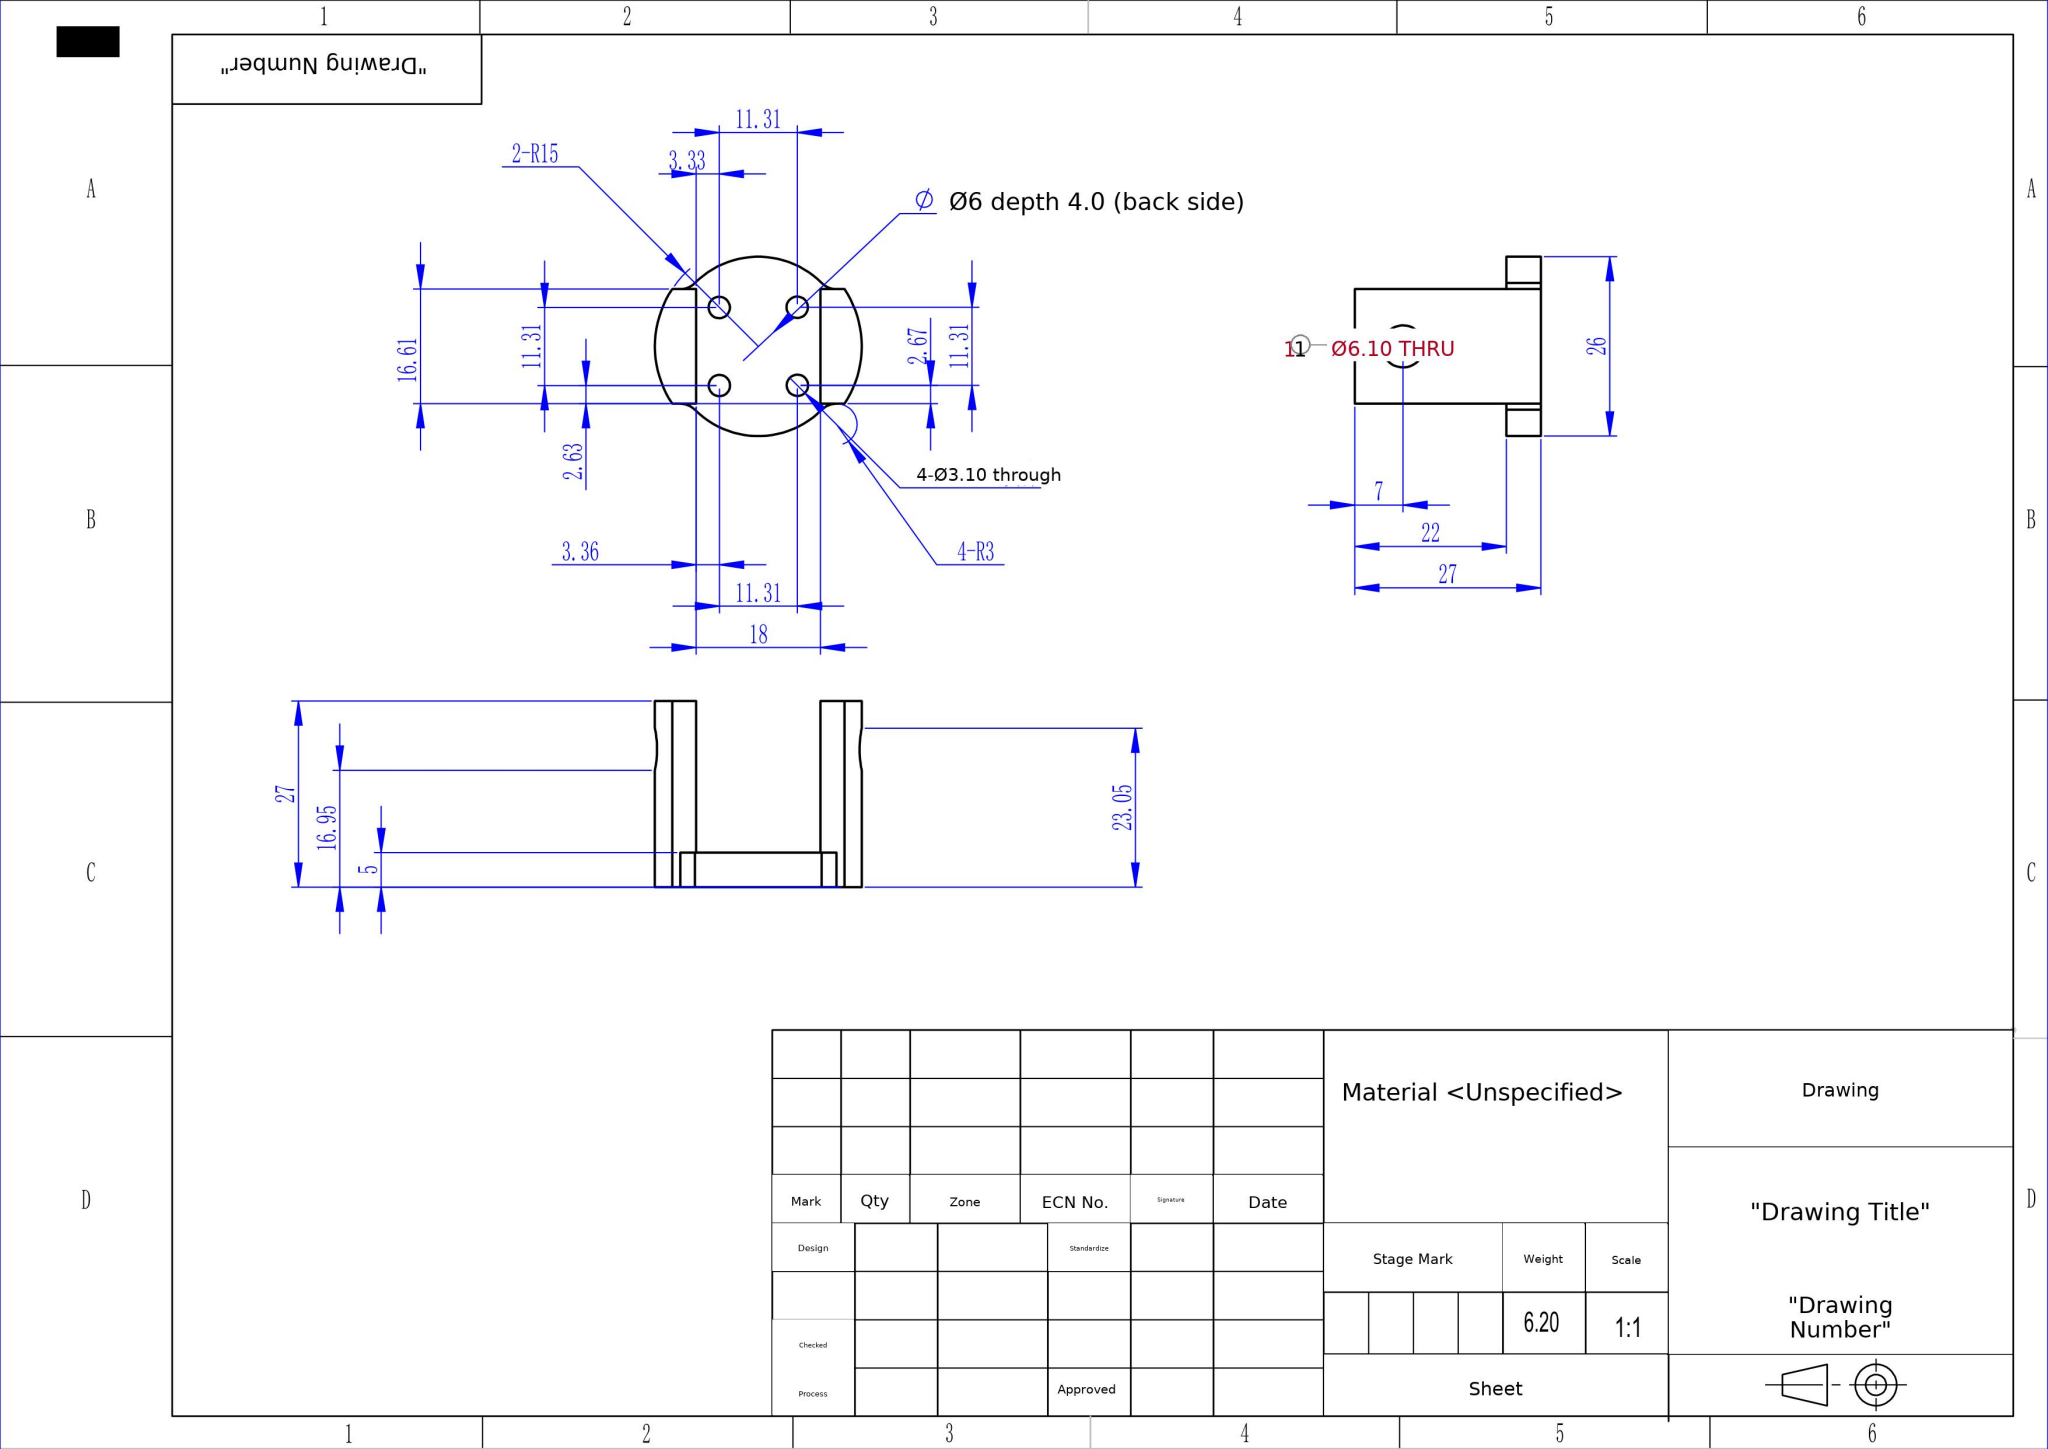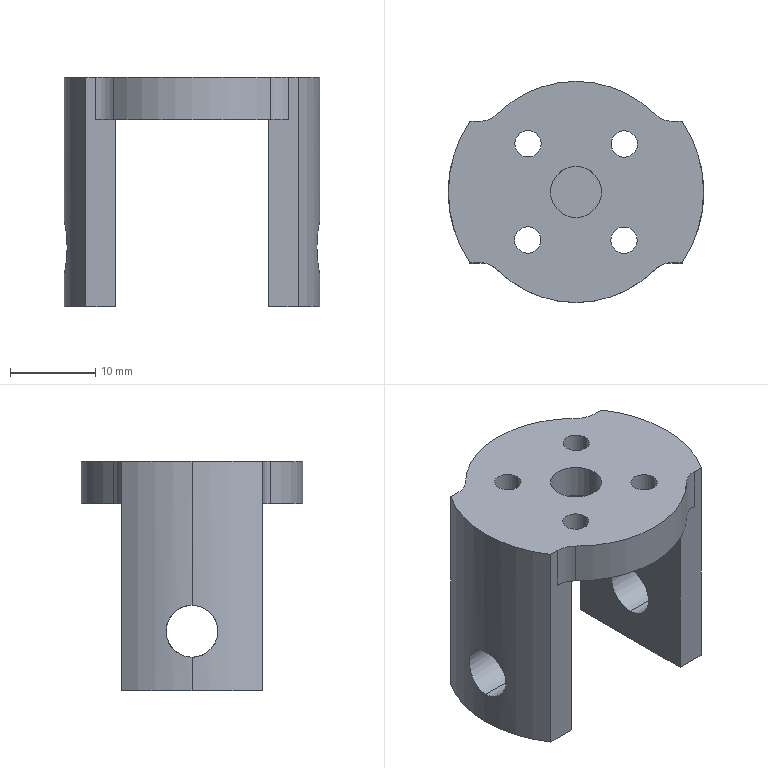Part | SolidWorks | mm | 1 solid | 34 faces | box 30 x 26 x 27 mm | volume 6201 mm3 | cylinder 23 | plane 11 | commonest cylinder face diameters 3.1 x8 6 x6 6.1 x4 30 x3 26 x2